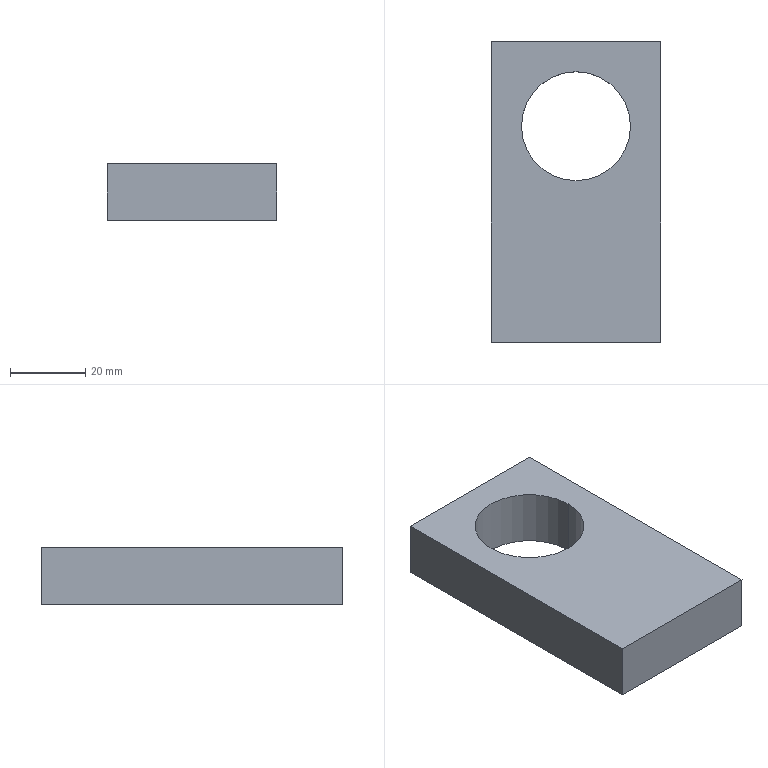Component | SolidWorks | HZ022-A001-E007-1 | 1 solid | 8 faces | box 45 x 80 x 15 mm | volume 44092 mm3 | plane 6 | cylinder 2 | commonest cylinder face diameters 29 x2 | material AL6061
build123d program:
from build123d import *

# Parameters (mm, degrees)
SKETCH1_W           = 80
SKETCH1_H           = 45
BOSS_EXTRUDE1_DEPTH = 15
SKETCH2_R           = 14.5
CUT_EXTRUDE1_DEPTH  = 49.283


with BuildPart() as part:
    # Sketch1 → Boss-Extrude1 (new body)
    with BuildSketch(Plane(origin=(0, 0, 0), x_dir=(1, 0, 0), z_dir=(0, 1, 0))):
        Rectangle(SKETCH1_W, SKETCH1_H)
    extrude(amount=BOSS_EXTRUDE1_DEPTH)

    # Sketch2 → Cut-Extrude1 (cut, through all)
    with BuildSketch(Plane(origin=(0, 15, 0), x_dir=(1, 0, 0), z_dir=(0, 1, 0))):
        with Locations(Location((17.5, 0, 0), (0, 0, 270))):
            Circle(SKETCH2_R)
    extrude(amount=-CUT_EXTRUDE1_DEPTH, mode=Mode.SUBTRACT)


solid = part.part

# Placed as in the assembly
solid = solid.moved(Location((198.244, 54.652, 784), (90, 90, 0)))
STEP:
#1=COLOUR_RGB('',0.7922,0.8196,0.9333);
#2=FILL_AREA_STYLE_COLOUR('',#1);
#3=FILL_AREA_STYLE('',(#2));
#4=SURFACE_STYLE_FILL_AREA(#3);
#5=SURFACE_SIDE_STYLE('',(#4));
#6=SURFACE_STYLE_USAGE(.BOTH.,#5);
#7=PRESENTATION_STYLE_ASSIGNMENT((#6));
#8=CARTESIAN_POINT('',(8.376,2.841,31.457));
#9=VERTEX_POINT('',#8);
#10=CARTESIAN_POINT('',(7.234,2.841,31.457));
#11=VERTEX_POINT('',#10);
#12=CARTESIAN_POINT('',(7.805,2.841,31.457));
#13=DIRECTION('',(-0.,0.,-1.));
#14=DIRECTION('',(-1.,0.,0.));
#15=AXIS2_PLACEMENT_3D('',#12,#13,#14);
#16=CIRCLE('',#15,0.5709);
#17=EDGE_CURVE('',#9,#11,#16,.T.);
#18=ORIENTED_EDGE('',*,*,#17,.F.);
#19=CARTESIAN_POINT('',(8.376,2.841,30.866));
#20=VERTEX_POINT('',#19);
#21=CARTESIAN_POINT('',(8.376,2.841,31.457));
#22=DIRECTION('',(-0.,0.,-1.));
#23=VECTOR('',#22,39.37);
#24=LINE('',#21,#23);
#25=EDGE_CURVE('',#9,#20,#24,.T.);
#26=ORIENTED_EDGE('',*,*,#25,.T.);
#27=CARTESIAN_POINT('',(7.234,2.841,30.866));
#28=VERTEX_POINT('',#27);
#29=CARTESIAN_POINT('',(7.805,2.841,30.866));
#30=DIRECTION('',(-0.,0.,-1.));
#31=DIRECTION('',(-1.,0.,0.));
#32=AXIS2_PLACEMENT_3D('',#29,#30,#31);
#33=CIRCLE('',#32,0.5709);
#34=EDGE_CURVE('',#20,#28,#33,.T.);
#35=ORIENTED_EDGE('',*,*,#34,.T.);
#36=CARTESIAN_POINT('',(7.234,2.841,31.457));
#37=DIRECTION('',(-0.,0.,-1.));
#38=VECTOR('',#37,39.37);
#39=LINE('',#36,#38);
#40=EDGE_CURVE('',#11,#28,#39,.T.);
#41=ORIENTED_EDGE('',*,*,#40,.F.);
#42=EDGE_LOOP('',(#18,#26,#35,#41));
#43=FACE_OUTER_BOUND('',#42,.T.);
#44=CARTESIAN_POINT('',(7.805,2.841,31.457));
#45=DIRECTION('',(-0.,0.,-1.));
#46=DIRECTION('',(-1.,0.,0.));
#47=AXIS2_PLACEMENT_3D('',#44,#45,#46);
#48=CYLINDRICAL_SURFACE('',#47,0.5709);
#49=ADVANCED_FACE('',(#43),#48,.F.);
#50=CARTESIAN_POINT('',(6.919,3.726,31.457));
#51=VERTEX_POINT('',#50);
#52=CARTESIAN_POINT('',(8.691,3.726,31.457));
#53=VERTEX_POINT('',#52);
#54=CARTESIAN_POINT('',(8.691,3.726,31.457));
#55=DIRECTION('',(1.,-0.,-0.));
#56=VECTOR('',#55,39.37);
#57=LINE('',#54,#56);
#58=EDGE_CURVE('',#51,#53,#57,.T.);
#59=ORIENTED_EDGE('',*,*,#58,.T.);
#60=CARTESIAN_POINT('',(8.691,3.726,30.866));
#61=VERTEX_POINT('',#60);
#62=CARTESIAN_POINT('',(8.691,3.726,30.866));
#63=DIRECTION('',(0.,0.,1.));
#64=VECTOR('',#63,39.37);
#65=LINE('',#62,#64);
#66=EDGE_CURVE('',#61,#53,#65,.T.);
#67=ORIENTED_EDGE('',*,*,#66,.F.);
#68=CARTESIAN_POINT('',(6.919,3.726,30.866));
#69=VERTEX_POINT('',#68);
#70=CARTESIAN_POINT('',(8.691,3.726,30.866));
#71=DIRECTION('',(1.,-0.,-0.));
#72=VECTOR('',#71,39.37);
#73=LINE('',#70,#72);
#74=EDGE_CURVE('',#69,#61,#73,.T.);
#75=ORIENTED_EDGE('',*,*,#74,.F.);
#76=CARTESIAN_POINT('',(6.919,3.726,30.866));
#77=DIRECTION('',(0.,0.,1.));
#78=VECTOR('',#77,39.37);
#79=LINE('',#76,#78);
#80=EDGE_CURVE('',#69,#51,#79,.T.);
#81=ORIENTED_EDGE('',*,*,#80,.T.);
#82=EDGE_LOOP('',(#59,#67,#75,#81));
#83=FACE_OUTER_BOUND('',#82,.T.);
#84=CARTESIAN_POINT('',(8.691,3.726,30.866));
#85=DIRECTION('',(-0.,-1.,0.));
#86=DIRECTION('',(-1.,0.,0.));
#87=AXIS2_PLACEMENT_3D('',#84,#85,#86);
#88=PLANE('',#87);
#89=ADVANCED_FACE('',(#83),#88,.F.);
#90=CARTESIAN_POINT('',(8.691,0.5769,31.457));
#91=VERTEX_POINT('',#90);
#92=CARTESIAN_POINT('',(8.691,0.5769,31.457));
#93=DIRECTION('',(-0.,-1.,0.));
#94=VECTOR('',#93,39.37);
#95=LINE('',#92,#94);
#96=EDGE_CURVE('',#53,#91,#95,.T.);
#97=ORIENTED_EDGE('',*,*,#96,.T.);
#98=CARTESIAN_POINT('',(8.691,0.5769,30.866));
#99=VERTEX_POINT('',#98);
#100=CARTESIAN_POINT('',(8.691,0.5769,30.866));
#101=DIRECTION('',(0.,0.,1.));
#102=VECTOR('',#101,39.37);
#103=LINE('',#100,#102);
#104=EDGE_CURVE('',#99,#91,#103,.T.);
#105=ORIENTED_EDGE('',*,*,#104,.F.);
#106=CARTESIAN_POINT('',(8.691,0.5769,30.866));
#107=DIRECTION('',(-0.,-1.,0.));
#108=VECTOR('',#107,39.37);
#109=LINE('',#106,#108);
#110=EDGE_CURVE('',#61,#99,#109,.T.);
#111=ORIENTED_EDGE('',*,*,#110,.F.);
#112=ORIENTED_EDGE('',*,*,#66,.T.);
#113=EDGE_LOOP('',(#97,#105,#111,#112));
#114=FACE_OUTER_BOUND('',#113,.T.);
#115=CARTESIAN_POINT('',(8.691,0.5769,30.866));
#116=DIRECTION('',(-1.,0.,0.));
#117=DIRECTION('',(0.,1.,0.));
#118=AXIS2_PLACEMENT_3D('',#115,#116,#117);
#119=PLANE('',#118);
#120=ADVANCED_FACE('',(#114),#119,.F.);
#121=CARTESIAN_POINT('',(6.919,0.5769,31.457));
#122=VERTEX_POINT('',#121);
#123=CARTESIAN_POINT('',(8.691,0.5769,31.457));
#124=DIRECTION('',(-1.,0.,0.));
#125=VECTOR('',#124,39.37);
#126=LINE('',#123,#125);
#127=EDGE_CURVE('',#91,#122,#126,.T.);
#128=ORIENTED_EDGE('',*,*,#127,.T.);
#129=CARTESIAN_POINT('',(6.919,0.5769,30.866));
#130=VERTEX_POINT('',#129);
#131=CARTESIAN_POINT('',(6.919,0.5769,30.866));
#132=DIRECTION('',(0.,0.,1.));
#133=VECTOR('',#132,39.37);
#134=LINE('',#131,#133);
#135=EDGE_CURVE('',#130,#122,#134,.T.);
#136=ORIENTED_EDGE('',*,*,#135,.F.);
#137=CARTESIAN_POINT('',(8.691,0.5769,30.866));
#138=DIRECTION('',(-1.,0.,0.));
#139=VECTOR('',#138,39.37);
#140=LINE('',#137,#139);
#141=EDGE_CURVE('',#99,#130,#140,.T.);
#142=ORIENTED_EDGE('',*,*,#141,.F.);
#143=ORIENTED_EDGE('',*,*,#104,.T.);
#144=EDGE_LOOP('',(#128,#136,#142,#143));
#145=FACE_OUTER_BOUND('',#144,.T.);
#146=CARTESIAN_POINT('',(8.691,0.5769,30.866));
#147=DIRECTION('',(0.,1.,-0.));
#148=DIRECTION('',(1.,-0.,-0.));
#149=AXIS2_PLACEMENT_3D('',#146,#147,#148);
#150=PLANE('',#149);
#151=ADVANCED_FACE('',(#145),#150,.F.);
#152=CARTESIAN_POINT('',(6.919,0.5769,31.457));
#153=DIRECTION('',(0.,1.,0.));
#154=VECTOR('',#153,39.37);
#155=LINE('',#152,#154);
#156=EDGE_CURVE('',#122,#51,#155,.T.);
#157=ORIENTED_EDGE('',*,*,#156,.T.);
#158=ORIENTED_EDGE('',*,*,#80,.F.);
#159=CARTESIAN_POINT('',(6.919,0.5769,30.866));
#160=DIRECTION('',(0.,1.,0.));
#161=VECTOR('',#160,39.37);
#162=LINE('',#159,#161);
#163=EDGE_CURVE('',#130,#69,#162,.T.);
#164=ORIENTED_EDGE('',*,*,#163,.F.);
#165=ORIENTED_EDGE('',*,*,#135,.T.);
#166=EDGE_LOOP('',(#157,#158,#164,#165));
#167=FACE_OUTER_BOUND('',#166,.T.);
#168=CARTESIAN_POINT('',(6.919,0.5769,30.866));
#169=DIRECTION('',(1.,-0.,-0.));
#170=DIRECTION('',(-0.,-1.,0.));
#171=AXIS2_PLACEMENT_3D('',#168,#169,#170);
#172=PLANE('',#171);
#173=ADVANCED_FACE('',(#167),#172,.F.);
#174=CARTESIAN_POINT('',(7.805,2.841,30.866));
#175=DIRECTION('',(-0.,0.,-1.));
#176=DIRECTION('',(-1.,0.,0.));
#177=AXIS2_PLACEMENT_3D('',#174,#175,#176);
#178=CIRCLE('',#177,0.5709);
#179=EDGE_CURVE('',#28,#20,#178,.T.);
#180=ORIENTED_EDGE('',*,*,#179,.F.);
#181=ORIENTED_EDGE('',*,*,#34,.F.);
#182=EDGE_LOOP('',(#180,#181));
#183=FACE_BOUND('',#182,.T.);
#184=ORIENTED_EDGE('',*,*,#74,.T.);
#185=ORIENTED_EDGE('',*,*,#110,.T.);
#186=ORIENTED_EDGE('',*,*,#141,.T.);
#187=ORIENTED_EDGE('',*,*,#163,.T.);
#188=EDGE_LOOP('',(#184,#185,#186,#187));
#189=FACE_OUTER_BOUND('',#188,.T.);
#190=CARTESIAN_POINT('',(7.805,2.152,30.866));
#191=DIRECTION('',(-0.,0.,-1.));
#192=DIRECTION('',(-1.,0.,0.));
#193=AXIS2_PLACEMENT_3D('',#190,#191,#192);
#194=PLANE('',#193);
#195=ADVANCED_FACE('',(#183,#189),#194,.T.);
#196=CARTESIAN_POINT('',(7.805,2.841,31.457));
#197=DIRECTION('',(-0.,0.,-1.));
#198=DIRECTION('',(-1.,0.,0.));
#199=AXIS2_PLACEMENT_3D('',#196,#197,#198);
#200=CIRCLE('',#199,0.5709);
#201=EDGE_CURVE('',#11,#9,#200,.T.);
#202=ORIENTED_EDGE('',*,*,#201,.T.);
#203=ORIENTED_EDGE('',*,*,#17,.T.);
#204=EDGE_LOOP('',(#202,#203));
#205=FACE_BOUND('',#204,.T.);
#206=ORIENTED_EDGE('',*,*,#58,.F.);
#207=ORIENTED_EDGE('',*,*,#156,.F.);
#208=ORIENTED_EDGE('',*,*,#127,.F.);
#209=ORIENTED_EDGE('',*,*,#96,.F.);
#210=EDGE_LOOP('',(#206,#207,#208,#209));
#211=FACE_OUTER_BOUND('',#210,.T.);
#212=CARTESIAN_POINT('',(7.805,2.152,31.457));
#213=DIRECTION('',(-0.,0.,-1.));
#214=DIRECTION('',(-1.,0.,0.));
#215=AXIS2_PLACEMENT_3D('',#212,#213,#214);
#216=PLANE('',#215);
#217=ADVANCED_FACE('',(#205,#211),#216,.F.);
#218=ORIENTED_EDGE('',*,*,#25,.F.);
#219=ORIENTED_EDGE('',*,*,#201,.F.);
#220=ORIENTED_EDGE('',*,*,#40,.T.);
#221=ORIENTED_EDGE('',*,*,#179,.T.);
#222=EDGE_LOOP('',(#218,#219,#220,#221));
#223=FACE_OUTER_BOUND('',#222,.T.);
#224=CARTESIAN_POINT('',(7.805,2.841,31.457));
#225=DIRECTION('',(-0.,0.,-1.));
#226=DIRECTION('',(-1.,0.,0.));
#227=AXIS2_PLACEMENT_3D('',#224,#225,#226);
#228=CYLINDRICAL_SURFACE('',#227,0.5709);
#229=ADVANCED_FACE('',(#223),#228,.F.);
#230=CLOSED_SHELL('',(#49,#89,#120,#151,#173,#195,#217,#229));
#231=MANIFOLD_SOLID_BREP('',#230);
#232=STYLED_ITEM('',(#7),#231);
#233=(LENGTH_UNIT()NAMED_UNIT(*)SI_UNIT($,.METRE.));
#234=LENGTH_MEASURE_WITH_UNIT(LENGTH_MEASURE(0.0254),#233);
#235=DIMENSIONAL_EXPONENTS(1.,0.,0.,0.,0.,0.,0.);
#236=(CONVERSION_BASED_UNIT('',#234)LENGTH_UNIT()NAMED_UNIT(#235));
#237=UNCERTAINTY_MEASURE_WITH_UNIT(LENGTH_MEASURE(0.00001),#236,'','');
#238=(NAMED_UNIT(*)PLANE_ANGLE_UNIT()SI_UNIT($,.RADIAN.));
#239=(NAMED_UNIT(*)SI_UNIT($,.STERADIAN.)SOLID_ANGLE_UNIT());
#240=(GEOMETRIC_REPRESENTATION_CONTEXT(3)GLOBAL_UNCERTAINTY_ASSIGNED_CONTEXT((#237))GLOBAL_UNIT_ASSIGNED_CONTEXT((#236,#238,#239))REPRESENTATION_CONTEXT('',''));
#241=MECHANICAL_DESIGN_GEOMETRIC_PRESENTATION_REPRESENTATION('',(#232),#240);
#242=CARTESIAN_POINT('',(0.,0.,0.));
#243=DIRECTION('',(0.,0.,1.));
#244=DIRECTION('',(1.,0.,0.));
#245=AXIS2_PLACEMENT_3D('',#242,#243,#244);
#246=(LENGTH_UNIT()NAMED_UNIT(*)SI_UNIT($,.METRE.));
#247=LENGTH_MEASURE_WITH_UNIT(LENGTH_MEASURE(0.0254),#246);
#248=DIMENSIONAL_EXPONENTS(1.,0.,0.,0.,0.,0.,0.);
#249=(CONVERSION_BASED_UNIT('',#247)LENGTH_UNIT()NAMED_UNIT(#248));
#250=UNCERTAINTY_MEASURE_WITH_UNIT(LENGTH_MEASURE(0.00001),#249,'','');
#251=(NAMED_UNIT(*)PLANE_ANGLE_UNIT()SI_UNIT($,.RADIAN.));
#252=(NAMED_UNIT(*)SI_UNIT($,.STERADIAN.)SOLID_ANGLE_UNIT());
#253=(GEOMETRIC_REPRESENTATION_CONTEXT(3)GLOBAL_UNCERTAINTY_ASSIGNED_CONTEXT((#250))GLOBAL_UNIT_ASSIGNED_CONTEXT((#249,#251,#252))REPRESENTATION_CONTEXT('',''));
#254=ADVANCED_BREP_SHAPE_REPRESENTATION('',(#231,#245),#253);
#255=PRESENTATION_LAYER_ASSIGNMENT('','',(#232));